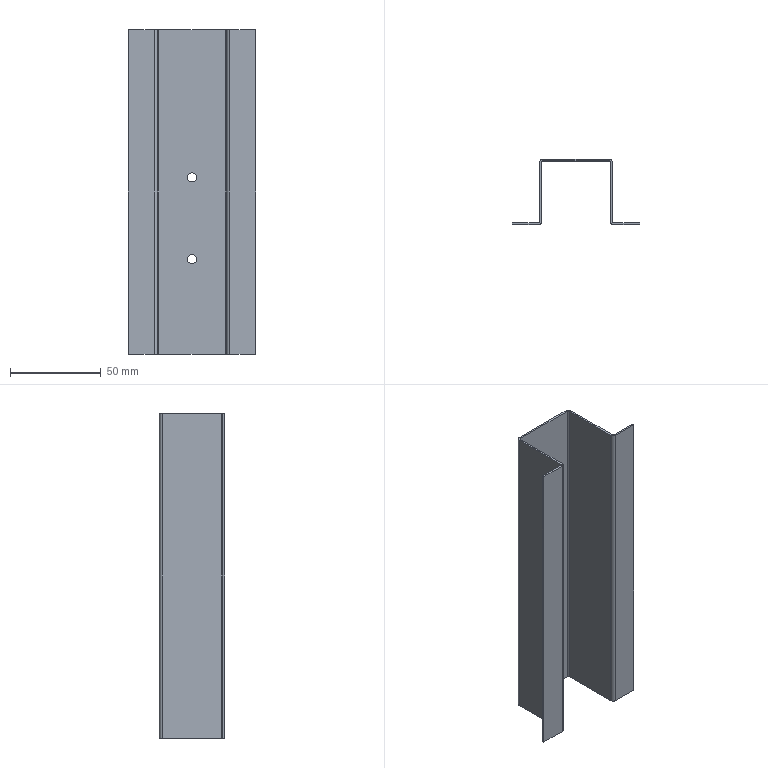Component | SolidWorks | CCQ-1.1-19Support1-1 | 1 solid | 34 faces | box 70 x 36 x 179 mm | volume 24641 mm3 | plane 22 | cylinder 12 | commonest cylinder face diameters 5 x4 1.473 x4 3.473 x4 | material 304
STEP:
#1=CARTESIAN_POINT('',(-2.067,-16.634,-3.327));
#2=VERTEX_POINT('',#1);
#3=CARTESIAN_POINT('',(-2.264,-16.634,-3.327));
#4=VERTEX_POINT('',#3);
#5=CARTESIAN_POINT('',(-2.165,-16.634,-3.327));
#6=DIRECTION('',(-0.,1.,0.));
#7=DIRECTION('',(-1.,0.,0.));
#8=AXIS2_PLACEMENT_3D('',#5,#6,#7);
#9=CIRCLE('',#8,0.09843);
#10=EDGE_CURVE('',#2,#4,#9,.T.);
#11=ORIENTED_EDGE('',*,*,#10,.F.);
#12=CARTESIAN_POINT('',(-2.067,-16.594,-3.327));
#13=VERTEX_POINT('',#12);
#14=CARTESIAN_POINT('',(-2.067,-16.988,-3.327));
#15=DIRECTION('',(-0.,1.,0.));
#16=VECTOR('',#15,39.37);
#17=LINE('',#14,#16);
#18=EDGE_CURVE('',#2,#13,#17,.T.);
#19=ORIENTED_EDGE('',*,*,#18,.T.);
#20=CARTESIAN_POINT('',(-2.264,-16.594,-3.327));
#21=VERTEX_POINT('',#20);
#22=CARTESIAN_POINT('',(-2.165,-16.594,-3.327));
#23=DIRECTION('',(-0.,1.,0.));
#24=DIRECTION('',(-1.,0.,0.));
#25=AXIS2_PLACEMENT_3D('',#22,#23,#24);
#26=CIRCLE('',#25,0.09843);
#27=EDGE_CURVE('',#13,#21,#26,.T.);
#28=ORIENTED_EDGE('',*,*,#27,.T.);
#29=CARTESIAN_POINT('',(-2.264,-16.988,-3.327));
#30=DIRECTION('',(-0.,1.,0.));
#31=VECTOR('',#30,39.37);
#32=LINE('',#29,#31);
#33=EDGE_CURVE('',#4,#21,#32,.T.);
#34=ORIENTED_EDGE('',*,*,#33,.F.);
#35=EDGE_LOOP('',(#11,#19,#28,#34));
#36=FACE_OUTER_BOUND('',#35,.T.);
#37=CARTESIAN_POINT('',(-2.165,-16.988,-3.327));
#38=DIRECTION('',(-0.,1.,0.));
#39=DIRECTION('',(-1.,0.,0.));
#40=AXIS2_PLACEMENT_3D('',#37,#38,#39);
#41=CYLINDRICAL_SURFACE('',#40,0.09843);
#42=ADVANCED_FACE('',(#36),#41,.F.);
#43=CARTESIAN_POINT('',(-2.067,-16.634,-5.098));
#44=VERTEX_POINT('',#43);
#45=CARTESIAN_POINT('',(-2.264,-16.634,-5.098));
#46=VERTEX_POINT('',#45);
#47=CARTESIAN_POINT('',(-2.165,-16.634,-5.098));
#48=DIRECTION('',(-0.,1.,0.));
#49=DIRECTION('',(-1.,0.,0.));
#50=AXIS2_PLACEMENT_3D('',#47,#48,#49);
#51=CIRCLE('',#50,0.09843);
#52=EDGE_CURVE('',#44,#46,#51,.T.);
#53=ORIENTED_EDGE('',*,*,#52,.F.);
#54=CARTESIAN_POINT('',(-2.067,-16.594,-5.098));
#55=VERTEX_POINT('',#54);
#56=CARTESIAN_POINT('',(-2.067,-16.988,-5.098));
#57=DIRECTION('',(-0.,1.,0.));
#58=VECTOR('',#57,39.37);
#59=LINE('',#56,#58);
#60=EDGE_CURVE('',#44,#55,#59,.T.);
#61=ORIENTED_EDGE('',*,*,#60,.T.);
#62=CARTESIAN_POINT('',(-2.264,-16.594,-5.098));
#63=VERTEX_POINT('',#62);
#64=CARTESIAN_POINT('',(-2.165,-16.594,-5.098));
#65=DIRECTION('',(-0.,1.,0.));
#66=DIRECTION('',(-1.,0.,0.));
#67=AXIS2_PLACEMENT_3D('',#64,#65,#66);
#68=CIRCLE('',#67,0.09843);
#69=EDGE_CURVE('',#55,#63,#68,.T.);
#70=ORIENTED_EDGE('',*,*,#69,.T.);
#71=CARTESIAN_POINT('',(-2.264,-16.988,-5.098));
#72=DIRECTION('',(-0.,1.,0.));
#73=VECTOR('',#72,39.37);
#74=LINE('',#71,#73);
#75=EDGE_CURVE('',#46,#63,#74,.T.);
#76=ORIENTED_EDGE('',*,*,#75,.F.);
#77=EDGE_LOOP('',(#53,#61,#70,#76));
#78=FACE_OUTER_BOUND('',#77,.T.);
#79=CARTESIAN_POINT('',(-2.165,-16.988,-5.098));
#80=DIRECTION('',(-0.,1.,0.));
#81=DIRECTION('',(-1.,0.,0.));
#82=AXIS2_PLACEMENT_3D('',#79,#80,#81);
#83=CYLINDRICAL_SURFACE('',#82,0.09843);
#84=ADVANCED_FACE('',(#78),#83,.F.);
#85=CARTESIAN_POINT('',(-2.982,-17.972,-7.165));
#86=VERTEX_POINT('',#85);
#87=CARTESIAN_POINT('',(-2.982,-18.012,-7.165));
#88=VERTEX_POINT('',#87);
#89=CARTESIAN_POINT('',(-2.982,-17.972,-7.165));
#90=DIRECTION('',(0.,-1.,0.));
#91=VECTOR('',#90,39.37);
#92=LINE('',#89,#91);
#93=EDGE_CURVE('',#86,#88,#92,.T.);
#94=ORIENTED_EDGE('',*,*,#93,.F.);
#95=CARTESIAN_POINT('',(-2.953,-17.943,-7.165));
#96=VERTEX_POINT('',#95);
#97=CARTESIAN_POINT('',(-2.982,-17.943,-7.165));
#98=DIRECTION('',(0.,0.,1.));
#99=DIRECTION('',(-1.,0.,0.));
#100=AXIS2_PLACEMENT_3D('',#97,#98,#99);
#101=CIRCLE('',#100,0.029);
#102=EDGE_CURVE('',#86,#96,#101,.T.);
#103=ORIENTED_EDGE('',*,*,#102,.T.);
#104=CARTESIAN_POINT('',(-2.913,-17.943,-7.165));
#105=VERTEX_POINT('',#104);
#106=CARTESIAN_POINT('',(-2.913,-17.943,-7.165));
#107=DIRECTION('',(-1.,0.,0.));
#108=VECTOR('',#107,39.37);
#109=LINE('',#106,#108);
#110=EDGE_CURVE('',#105,#96,#109,.T.);
#111=ORIENTED_EDGE('',*,*,#110,.F.);
#112=CARTESIAN_POINT('',(-2.982,-17.943,-7.165));
#113=DIRECTION('',(0.,0.,1.));
#114=DIRECTION('',(1.,0.,0.));
#115=AXIS2_PLACEMENT_3D('',#112,#113,#114);
#116=CIRCLE('',#115,0.06837);
#117=EDGE_CURVE('',#88,#105,#116,.T.);
#118=ORIENTED_EDGE('',*,*,#117,.F.);
#119=EDGE_LOOP('',(#94,#103,#111,#118));
#120=FACE_OUTER_BOUND('',#119,.T.);
#121=CARTESIAN_POINT('',(-2.982,-17.972,-7.165));
#122=DIRECTION('',(0.,0.,-1.));
#123=DIRECTION('',(-1.,0.,0.));
#124=AXIS2_PLACEMENT_3D('',#121,#122,#123);
#125=PLANE('',#124);
#126=ADVANCED_FACE('',(#120),#125,.T.);
#127=CARTESIAN_POINT('',(-3.543,-17.972,-7.165));
#128=VERTEX_POINT('',#127);
#129=CARTESIAN_POINT('',(-3.543,-17.972,-7.165));
#130=DIRECTION('',(1.,0.,0.));
#131=VECTOR('',#130,39.37);
#132=LINE('',#129,#131);
#133=EDGE_CURVE('',#128,#86,#132,.T.);
#134=ORIENTED_EDGE('',*,*,#133,.T.);
#135=ORIENTED_EDGE('',*,*,#93,.T.);
#136=CARTESIAN_POINT('',(-3.543,-18.012,-7.165));
#137=VERTEX_POINT('',#136);
#138=CARTESIAN_POINT('',(-3.543,-18.012,-7.165));
#139=DIRECTION('',(1.,0.,0.));
#140=VECTOR('',#139,39.37);
#141=LINE('',#138,#140);
#142=EDGE_CURVE('',#137,#88,#141,.T.);
#143=ORIENTED_EDGE('',*,*,#142,.F.);
#144=CARTESIAN_POINT('',(-3.543,-18.012,-7.165));
#145=DIRECTION('',(0.,1.,0.));
#146=VECTOR('',#145,39.37);
#147=LINE('',#144,#146);
#148=EDGE_CURVE('',#137,#128,#147,.T.);
#149=ORIENTED_EDGE('',*,*,#148,.T.);
#150=EDGE_LOOP('',(#134,#135,#143,#149));
#151=FACE_OUTER_BOUND('',#150,.T.);
#152=CARTESIAN_POINT('',(-2.913,-17.943,-7.165));
#153=DIRECTION('',(0.,0.,-1.));
#154=DIRECTION('',(-1.,0.,0.));
#155=AXIS2_PLACEMENT_3D('',#152,#153,#154);
#156=PLANE('',#155);
#157=ADVANCED_FACE('',(#151),#156,.T.);
#158=CARTESIAN_POINT('',(-2.953,-16.663,-7.165));
#159=VERTEX_POINT('',#158);
#160=CARTESIAN_POINT('',(-2.913,-16.663,-7.165));
#161=VERTEX_POINT('',#160);
#162=CARTESIAN_POINT('',(-2.953,-16.663,-7.165));
#163=DIRECTION('',(1.,0.,0.));
#164=VECTOR('',#163,39.37);
#165=LINE('',#162,#164);
#166=EDGE_CURVE('',#159,#161,#165,.T.);
#167=ORIENTED_EDGE('',*,*,#166,.F.);
#168=CARTESIAN_POINT('',(-2.884,-16.594,-7.165));
#169=VERTEX_POINT('',#168);
#170=CARTESIAN_POINT('',(-2.884,-16.663,-7.165));
#171=DIRECTION('',(0.,0.,-1.));
#172=DIRECTION('',(1.,0.,0.));
#173=AXIS2_PLACEMENT_3D('',#170,#171,#172);
#174=CIRCLE('',#173,0.06837);
#175=EDGE_CURVE('',#159,#169,#174,.T.);
#176=ORIENTED_EDGE('',*,*,#175,.T.);
#177=CARTESIAN_POINT('',(-2.884,-16.634,-7.165));
#178=VERTEX_POINT('',#177);
#179=CARTESIAN_POINT('',(-2.884,-16.634,-7.165));
#180=DIRECTION('',(0.,1.,0.));
#181=VECTOR('',#180,39.37);
#182=LINE('',#179,#181);
#183=EDGE_CURVE('',#178,#169,#182,.T.);
#184=ORIENTED_EDGE('',*,*,#183,.F.);
#185=CARTESIAN_POINT('',(-2.884,-16.663,-7.165));
#186=DIRECTION('',(0.,0.,-1.));
#187=DIRECTION('',(1.,0.,0.));
#188=AXIS2_PLACEMENT_3D('',#185,#186,#187);
#189=CIRCLE('',#188,0.029);
#190=EDGE_CURVE('',#161,#178,#189,.T.);
#191=ORIENTED_EDGE('',*,*,#190,.F.);
#192=EDGE_LOOP('',(#167,#176,#184,#191));
#193=FACE_OUTER_BOUND('',#192,.T.);
#194=CARTESIAN_POINT('',(-2.953,-16.663,-7.165));
#195=DIRECTION('',(0.,0.,-1.));
#196=DIRECTION('',(-1.,0.,0.));
#197=AXIS2_PLACEMENT_3D('',#194,#195,#196);
#198=PLANE('',#197);
#199=ADVANCED_FACE('',(#193),#198,.T.);
#200=CARTESIAN_POINT('',(-2.953,-17.972,-7.165));
#201=DIRECTION('',(0.,1.,0.));
#202=VECTOR('',#201,39.37);
#203=LINE('',#200,#202);
#204=EDGE_CURVE('',#96,#159,#203,.T.);
#205=ORIENTED_EDGE('',*,*,#204,.T.);
#206=ORIENTED_EDGE('',*,*,#166,.T.);
#207=CARTESIAN_POINT('',(-2.913,-17.972,-7.165));
#208=DIRECTION('',(0.,1.,0.));
#209=VECTOR('',#208,39.37);
#210=LINE('',#207,#209);
#211=EDGE_CURVE('',#105,#161,#210,.T.);
#212=ORIENTED_EDGE('',*,*,#211,.F.);
#213=ORIENTED_EDGE('',*,*,#110,.T.);
#214=EDGE_LOOP('',(#205,#206,#212,#213));
#215=FACE_OUTER_BOUND('',#214,.T.);
#216=CARTESIAN_POINT('',(-2.884,-16.634,-7.165));
#217=DIRECTION('',(0.,0.,-1.));
#218=DIRECTION('',(-1.,0.,0.));
#219=AXIS2_PLACEMENT_3D('',#216,#217,#218);
#220=PLANE('',#219);
#221=ADVANCED_FACE('',(#215),#220,.T.);
#222=CARTESIAN_POINT('',(-1.446,-16.594,-7.165));
#223=VERTEX_POINT('',#222);
#224=CARTESIAN_POINT('',(-1.446,-16.634,-7.165));
#225=VERTEX_POINT('',#224);
#226=CARTESIAN_POINT('',(-1.446,-16.594,-7.165));
#227=DIRECTION('',(0.,-1.,0.));
#228=VECTOR('',#227,39.37);
#229=LINE('',#226,#228);
#230=EDGE_CURVE('',#223,#225,#229,.T.);
#231=ORIENTED_EDGE('',*,*,#230,.F.);
#232=CARTESIAN_POINT('',(-1.378,-16.663,-7.165));
#233=VERTEX_POINT('',#232);
#234=CARTESIAN_POINT('',(-1.446,-16.663,-7.165));
#235=DIRECTION('',(0.,0.,-1.));
#236=DIRECTION('',(1.,0.,0.));
#237=AXIS2_PLACEMENT_3D('',#234,#235,#236);
#238=CIRCLE('',#237,0.06837);
#239=EDGE_CURVE('',#223,#233,#238,.T.);
#240=ORIENTED_EDGE('',*,*,#239,.T.);
#241=CARTESIAN_POINT('',(-1.417,-16.663,-7.165));
#242=VERTEX_POINT('',#241);
#243=CARTESIAN_POINT('',(-1.417,-16.663,-7.165));
#244=DIRECTION('',(1.,0.,0.));
#245=VECTOR('',#244,39.37);
#246=LINE('',#243,#245);
#247=EDGE_CURVE('',#242,#233,#246,.T.);
#248=ORIENTED_EDGE('',*,*,#247,.F.);
#249=CARTESIAN_POINT('',(-1.446,-16.663,-7.165));
#250=DIRECTION('',(0.,0.,-1.));
#251=DIRECTION('',(1.,0.,0.));
#252=AXIS2_PLACEMENT_3D('',#249,#250,#251);
#253=CIRCLE('',#252,0.029);
#254=EDGE_CURVE('',#225,#242,#253,.T.);
#255=ORIENTED_EDGE('',*,*,#254,.F.);
#256=EDGE_LOOP('',(#231,#240,#248,#255));
#257=FACE_OUTER_BOUND('',#256,.T.);
#258=CARTESIAN_POINT('',(-1.446,-16.594,-7.165));
#259=DIRECTION('',(0.,0.,-1.));
#260=DIRECTION('',(-1.,0.,0.));
#261=AXIS2_PLACEMENT_3D('',#258,#259,#260);
#262=PLANE('',#261);
#263=ADVANCED_FACE('',(#257),#262,.T.);
#264=CARTESIAN_POINT('',(-2.953,-16.594,-7.165));
#265=DIRECTION('',(1.,0.,0.));
#266=VECTOR('',#265,39.37);
#267=LINE('',#264,#266);
#268=EDGE_CURVE('',#169,#223,#267,.T.);
#269=ORIENTED_EDGE('',*,*,#268,.T.);
#270=ORIENTED_EDGE('',*,*,#230,.T.);
#271=CARTESIAN_POINT('',(-2.953,-16.634,-7.165));
#272=DIRECTION('',(1.,0.,0.));
#273=VECTOR('',#272,39.37);
#274=LINE('',#271,#273);
#275=EDGE_CURVE('',#178,#225,#274,.T.);
#276=ORIENTED_EDGE('',*,*,#275,.F.);
#277=ORIENTED_EDGE('',*,*,#183,.T.);
#278=EDGE_LOOP('',(#269,#270,#276,#277));
#279=FACE_OUTER_BOUND('',#278,.T.);
#280=CARTESIAN_POINT('',(-1.417,-16.663,-7.165));
#281=DIRECTION('',(0.,0.,-1.));
#282=DIRECTION('',(-1.,0.,0.));
#283=AXIS2_PLACEMENT_3D('',#280,#281,#282);
#284=PLANE('',#283);
#285=ADVANCED_FACE('',(#279),#284,.T.);
#286=CARTESIAN_POINT('',(-1.378,-17.943,-7.165));
#287=VERTEX_POINT('',#286);
#288=CARTESIAN_POINT('',(-1.417,-17.943,-7.165));
#289=VERTEX_POINT('',#288);
#290=CARTESIAN_POINT('',(-1.378,-17.943,-7.165));
#291=DIRECTION('',(-1.,-0.,0.));
#292=VECTOR('',#291,39.37);
#293=LINE('',#290,#292);
#294=EDGE_CURVE('',#287,#289,#293,.T.);
#295=ORIENTED_EDGE('',*,*,#294,.F.);
#296=CARTESIAN_POINT('',(-1.349,-17.972,-7.165));
#297=VERTEX_POINT('',#296);
#298=CARTESIAN_POINT('',(-1.349,-17.943,-7.165));
#299=DIRECTION('',(0.,0.,1.));
#300=DIRECTION('',(-1.,-0.,0.));
#301=AXIS2_PLACEMENT_3D('',#298,#299,#300);
#302=CIRCLE('',#301,0.029);
#303=EDGE_CURVE('',#287,#297,#302,.T.);
#304=ORIENTED_EDGE('',*,*,#303,.T.);
#305=CARTESIAN_POINT('',(-1.349,-18.012,-7.165));
#306=VERTEX_POINT('',#305);
#307=CARTESIAN_POINT('',(-1.349,-18.012,-7.165));
#308=DIRECTION('',(0.,1.,0.));
#309=VECTOR('',#308,39.37);
#310=LINE('',#307,#309);
#311=EDGE_CURVE('',#306,#297,#310,.T.);
#312=ORIENTED_EDGE('',*,*,#311,.F.);
#313=CARTESIAN_POINT('',(-1.349,-17.943,-7.165));
#314=DIRECTION('',(0.,0.,1.));
#315=DIRECTION('',(1.,0.,0.));
#316=AXIS2_PLACEMENT_3D('',#313,#314,#315);
#317=CIRCLE('',#316,0.06837);
#318=EDGE_CURVE('',#289,#306,#317,.T.);
#319=ORIENTED_EDGE('',*,*,#318,.F.);
#320=EDGE_LOOP('',(#295,#304,#312,#319));
#321=FACE_OUTER_BOUND('',#320,.T.);
#322=CARTESIAN_POINT('',(-1.378,-17.943,-7.165));
#323=DIRECTION('',(0.,0.,-1.));
#324=DIRECTION('',(-1.,0.,0.));
#325=AXIS2_PLACEMENT_3D('',#322,#323,#324);
#326=PLANE('',#325);
#327=ADVANCED_FACE('',(#321),#326,.T.);
#328=CARTESIAN_POINT('',(-1.378,-16.594,-7.165));
#329=DIRECTION('',(0.,-1.,0.));
#330=VECTOR('',#329,39.37);
#331=LINE('',#328,#330);
#332=EDGE_CURVE('',#233,#287,#331,.T.);
#333=ORIENTED_EDGE('',*,*,#332,.T.);
#334=ORIENTED_EDGE('',*,*,#294,.T.);
#335=CARTESIAN_POINT('',(-1.417,-16.594,-7.165));
#336=DIRECTION('',(0.,-1.,0.));
#337=VECTOR('',#336,39.37);
#338=LINE('',#335,#337);
#339=EDGE_CURVE('',#242,#289,#338,.T.);
#340=ORIENTED_EDGE('',*,*,#339,.F.);
#341=ORIENTED_EDGE('',*,*,#247,.T.);
#342=EDGE_LOOP('',(#333,#334,#340,#341));
#343=FACE_OUTER_BOUND('',#342,.T.);
#344=CARTESIAN_POINT('',(-1.349,-18.012,-7.165));
#345=DIRECTION('',(0.,0.,-1.));
#346=DIRECTION('',(-1.,0.,0.));
#347=AXIS2_PLACEMENT_3D('',#344,#345,#346);
#348=PLANE('',#347);
#349=ADVANCED_FACE('',(#343),#348,.T.);
#350=CARTESIAN_POINT('',(-0.7874,-18.012,-0.1181));
#351=VERTEX_POINT('',#350);
#352=CARTESIAN_POINT('',(-0.7874,-18.012,-7.165));
#353=VERTEX_POINT('',#352);
#354=CARTESIAN_POINT('',(-0.7874,-18.012,-0.07874));
#355=DIRECTION('',(0.,0.,-1.));
#356=VECTOR('',#355,39.37);
#357=LINE('',#354,#356);
#358=EDGE_CURVE('',#351,#353,#357,.T.);
#359=ORIENTED_EDGE('',*,*,#358,.F.);
#360=CARTESIAN_POINT('',(-1.349,-18.012,-0.1181));
#361=VERTEX_POINT('',#360);
#362=CARTESIAN_POINT('',(-1.378,-18.012,-0.1181));
#363=DIRECTION('',(-1.,0.,0.));
#364=VECTOR('',#363,39.37);
#365=LINE('',#362,#364);
#366=EDGE_CURVE('',#351,#361,#365,.T.);
#367=ORIENTED_EDGE('',*,*,#366,.T.);
#368=CARTESIAN_POINT('',(-1.349,-18.012,-0.07874));
#369=DIRECTION('',(0.,0.,-1.));
#370=VECTOR('',#369,39.37);
#371=LINE('',#368,#370);
#372=EDGE_CURVE('',#361,#306,#371,.T.);
#373=ORIENTED_EDGE('',*,*,#372,.T.);
#374=CARTESIAN_POINT('',(-1.378,-18.012,-7.165));
#375=DIRECTION('',(1.,-0.,0.));
#376=VECTOR('',#375,39.37);
#377=LINE('',#374,#376);
#378=EDGE_CURVE('',#306,#353,#377,.T.);
#379=ORIENTED_EDGE('',*,*,#378,.T.);
#380=EDGE_LOOP('',(#359,#367,#373,#379));
#381=FACE_OUTER_BOUND('',#380,.T.);
#382=CARTESIAN_POINT('',(-1.378,-18.012,-0.07874));
#383=DIRECTION('',(0.,1.,0.));
#384=DIRECTION('',(-1.,0.,0.));
#385=AXIS2_PLACEMENT_3D('',#382,#383,#384);
#386=PLANE('',#385);
#387=ADVANCED_FACE('',(#381),#386,.F.);
#388=CARTESIAN_POINT('',(-0.7874,-17.972,-0.1181));
#389=VERTEX_POINT('',#388);
#390=CARTESIAN_POINT('',(-0.7874,-17.972,-0.1181));
#391=DIRECTION('',(0.,1.,0.));
#392=VECTOR('',#391,39.37);
#393=LINE('',#390,#392);
#394=EDGE_CURVE('',#351,#389,#393,.T.);
#395=ORIENTED_EDGE('',*,*,#394,.F.);
#396=ORIENTED_EDGE('',*,*,#358,.T.);
#397=CARTESIAN_POINT('',(-0.7874,-17.972,-7.165));
#398=VERTEX_POINT('',#397);
#399=CARTESIAN_POINT('',(-0.7874,-17.972,-7.165));
#400=DIRECTION('',(0.,-1.,0.));
#401=VECTOR('',#400,39.37);
#402=LINE('',#399,#401);
#403=EDGE_CURVE('',#398,#353,#402,.T.);
#404=ORIENTED_EDGE('',*,*,#403,.F.);
#405=CARTESIAN_POINT('',(-0.7874,-17.972,-0.07874));
#406=DIRECTION('',(0.,0.,-1.));
#407=VECTOR('',#406,39.37);
#408=LINE('',#405,#407);
#409=EDGE_CURVE('',#389,#398,#408,.T.);
#410=ORIENTED_EDGE('',*,*,#409,.F.);
#411=EDGE_LOOP('',(#395,#396,#404,#410));
#412=FACE_OUTER_BOUND('',#411,.T.);
#413=CARTESIAN_POINT('',(-0.7874,-17.972,-0.07874));
#414=DIRECTION('',(1.,0.,0.));
#415=DIRECTION('',(0.,0.,-1.));
#416=AXIS2_PLACEMENT_3D('',#413,#414,#415);
#417=PLANE('',#416);
#418=ADVANCED_FACE('',(#412),#417,.T.);
#419=CARTESIAN_POINT('',(-1.349,-17.972,-0.1181));
#420=VERTEX_POINT('',#419);
#421=CARTESIAN_POINT('',(-1.378,-17.972,-0.1181));
#422=DIRECTION('',(-1.,0.,0.));
#423=VECTOR('',#422,39.37);
#424=LINE('',#421,#423);
#425=EDGE_CURVE('',#389,#420,#424,.T.);
#426=ORIENTED_EDGE('',*,*,#425,.F.);
#427=ORIENTED_EDGE('',*,*,#409,.T.);
#428=CARTESIAN_POINT('',(-1.378,-17.972,-7.165));
#429=DIRECTION('',(1.,-0.,0.));
#430=VECTOR('',#429,39.37);
#431=LINE('',#428,#430);
#432=EDGE_CURVE('',#297,#398,#431,.T.);
#433=ORIENTED_EDGE('',*,*,#432,.F.);
#434=CARTESIAN_POINT('',(-1.349,-17.972,-0.07874));
#435=DIRECTION('',(0.,0.,-1.));
#436=VECTOR('',#435,39.37);
#437=LINE('',#434,#436);
#438=EDGE_CURVE('',#420,#297,#437,.T.);
#439=ORIENTED_EDGE('',*,*,#438,.F.);
#440=EDGE_LOOP('',(#426,#427,#433,#439));
#441=FACE_OUTER_BOUND('',#440,.T.);
#442=CARTESIAN_POINT('',(-1.378,-17.972,-0.07874));
#443=DIRECTION('',(0.,1.,0.));
#444=DIRECTION('',(-1.,0.,0.));
#445=AXIS2_PLACEMENT_3D('',#442,#443,#444);
#446=PLANE('',#445);
#447=ADVANCED_FACE('',(#441),#446,.T.);
#448=CARTESIAN_POINT('',(-1.378,-17.943,-0.1181));
#449=VERTEX_POINT('',#448);
#450=CARTESIAN_POINT('',(-1.349,-17.943,-0.1181));
#451=DIRECTION('',(0.,0.,-1.));
#452=DIRECTION('',(-1.,0.,0.));
#453=AXIS2_PLACEMENT_3D('',#450,#451,#452);
#454=CIRCLE('',#453,0.029);
#455=EDGE_CURVE('',#420,#449,#454,.T.);
#456=ORIENTED_EDGE('',*,*,#455,.F.);
#457=ORIENTED_EDGE('',*,*,#438,.T.);
#458=ORIENTED_EDGE('',*,*,#303,.F.);
#459=CARTESIAN_POINT('',(-1.378,-17.943,-0.07874));
#460=DIRECTION('',(0.,0.,-1.));
#461=VECTOR('',#460,39.37);
#462=LINE('',#459,#461);
#463=EDGE_CURVE('',#449,#287,#462,.T.);
#464=ORIENTED_EDGE('',*,*,#463,.F.);
#465=EDGE_LOOP('',(#456,#457,#458,#464));
#466=FACE_OUTER_BOUND('',#465,.T.);
#467=CARTESIAN_POINT('',(-1.349,-17.943,-0.07874));
#468=DIRECTION('',(0.,0.,-1.));
#469=DIRECTION('',(-1.,0.,0.));
#470=AXIS2_PLACEMENT_3D('',#467,#468,#469);
#471=CYLINDRICAL_SURFACE('',#470,0.029);
#472=ADVANCED_FACE('',(#466),#471,.F.);
#473=CARTESIAN_POINT('',(-1.378,-16.663,-0.1181));
#474=VERTEX_POINT('',#473);
#475=CARTESIAN_POINT('',(-1.378,-16.594,-0.1181));
#476=DIRECTION('',(-0.,1.,0.));
#477=VECTOR('',#476,39.37);
#478=LINE('',#475,#477);
#479=EDGE_CURVE('',#449,#474,#478,.T.);
#480=ORIENTED_EDGE('',*,*,#479,.F.);
#481=ORIENTED_EDGE('',*,*,#463,.T.);
#482=ORIENTED_EDGE('',*,*,#332,.F.);
#483=CARTESIAN_POINT('',(-1.378,-16.663,-0.07874));
#484=DIRECTION('',(0.,0.,-1.));
#485=VECTOR('',#484,39.37);
#486=LINE('',#483,#485);
#487=EDGE_CURVE('',#474,#233,#486,.T.);
#488=ORIENTED_EDGE('',*,*,#487,.F.);
#489=EDGE_LOOP('',(#480,#481,#482,#488));
#490=FACE_OUTER_BOUND('',#489,.T.);
#491=CARTESIAN_POINT('',(-1.378,-16.594,-0.07874));
#492=DIRECTION('',(1.,0.,0.));
#493=DIRECTION('',(-0.,1.,0.));
#494=AXIS2_PLACEMENT_3D('',#491,#492,#493);
#495=PLANE('',#494);
#496=ADVANCED_FACE('',(#490),#495,.T.);
#497=CARTESIAN_POINT('',(-1.446,-16.594,-0.1181));
#498=VERTEX_POINT('',#497);
#499=CARTESIAN_POINT('',(-1.446,-16.663,-0.1181));
#500=DIRECTION('',(0.,0.,1.));
#501=DIRECTION('',(-1.,0.,0.));
#502=AXIS2_PLACEMENT_3D('',#499,#500,#501);
#503=CIRCLE('',#502,0.06837);
#504=EDGE_CURVE('',#474,#498,#503,.T.);
#505=ORIENTED_EDGE('',*,*,#504,.F.);
#506=ORIENTED_EDGE('',*,*,#487,.T.);
#507=ORIENTED_EDGE('',*,*,#239,.F.);
#508=CARTESIAN_POINT('',(-1.446,-16.594,-0.07874));
#509=DIRECTION('',(0.,0.,-1.));
#510=VECTOR('',#509,39.37);
#511=LINE('',#508,#510);
#512=EDGE_CURVE('',#498,#223,#511,.T.);
#513=ORIENTED_EDGE('',*,*,#512,.F.);
#514=EDGE_LOOP('',(#505,#506,#507,#513));
#515=FACE_OUTER_BOUND('',#514,.T.);
#516=CARTESIAN_POINT('',(-1.446,-16.663,-0.07874));
#517=DIRECTION('',(0.,0.,-1.));
#518=DIRECTION('',(-1.,0.,0.));
#519=AXIS2_PLACEMENT_3D('',#516,#517,#518);
#520=CYLINDRICAL_SURFACE('',#519,0.06837);
#521=ADVANCED_FACE('',(#515),#520,.T.);
#522=CARTESIAN_POINT('',(-2.884,-16.594,-0.1181));
#523=VERTEX_POINT('',#522);
#524=CARTESIAN_POINT('',(-2.953,-16.594,-0.1181));
#525=DIRECTION('',(-1.,-0.,0.));
#526=VECTOR('',#525,39.37);
#527=LINE('',#524,#526);
#528=EDGE_CURVE('',#498,#523,#527,.T.);
#529=ORIENTED_EDGE('',*,*,#528,.F.);
#530=ORIENTED_EDGE('',*,*,#512,.T.);
#531=ORIENTED_EDGE('',*,*,#268,.F.);
#532=CARTESIAN_POINT('',(-2.884,-16.594,-0.07874));
#533=DIRECTION('',(0.,0.,-1.));
#534=VECTOR('',#533,39.37);
#535=LINE('',#532,#534);
#536=EDGE_CURVE('',#523,#169,#535,.T.);
#537=ORIENTED_EDGE('',*,*,#536,.F.);
#538=EDGE_LOOP('',(#529,#530,#531,#537));
#539=FACE_OUTER_BOUND('',#538,.T.);
#540=CARTESIAN_POINT('',(-2.165,-16.594,-3.327));
#541=DIRECTION('',(-0.,1.,0.));
#542=DIRECTION('',(-1.,0.,0.));
#543=AXIS2_PLACEMENT_3D('',#540,#541,#542);
#544=CIRCLE('',#543,0.09843);
#545=EDGE_CURVE('',#21,#13,#544,.T.);
#546=ORIENTED_EDGE('',*,*,#545,.F.);
#547=ORIENTED_EDGE('',*,*,#27,.F.);
#548=EDGE_LOOP('',(#546,#547));
#549=FACE_BOUND('',#548,.T.);
#550=CARTESIAN_POINT('',(-2.165,-16.594,-5.098));
#551=DIRECTION('',(-0.,1.,0.));
#552=DIRECTION('',(-1.,0.,0.));
#553=AXIS2_PLACEMENT_3D('',#550,#551,#552);
#554=CIRCLE('',#553,0.09843);
#555=EDGE_CURVE('',#63,#55,#554,.T.);
#556=ORIENTED_EDGE('',*,*,#555,.F.);
#557=ORIENTED_EDGE('',*,*,#69,.F.);
#558=EDGE_LOOP('',(#556,#557));
#559=FACE_BOUND('',#558,.T.);
#560=CARTESIAN_POINT('',(-2.953,-16.594,-0.07874));
#561=DIRECTION('',(-0.,1.,0.));
#562=DIRECTION('',(-1.,-0.,0.));
#563=AXIS2_PLACEMENT_3D('',#560,#561,#562);
#564=PLANE('',#563);
#565=ADVANCED_FACE('',(#539,#549,#559),#564,.T.);
#566=CARTESIAN_POINT('',(-2.953,-16.663,-0.1181));
#567=VERTEX_POINT('',#566);
#568=CARTESIAN_POINT('',(-2.884,-16.663,-0.1181));
#569=DIRECTION('',(0.,0.,1.));
#570=DIRECTION('',(-1.,0.,0.));
#571=AXIS2_PLACEMENT_3D('',#568,#569,#570);
#572=CIRCLE('',#571,0.06837);
#573=EDGE_CURVE('',#523,#567,#572,.T.);
#574=ORIENTED_EDGE('',*,*,#573,.F.);
#575=ORIENTED_EDGE('',*,*,#536,.T.);
#576=ORIENTED_EDGE('',*,*,#175,.F.);
#577=CARTESIAN_POINT('',(-2.953,-16.663,-0.07874));
#578=DIRECTION('',(0.,0.,-1.));
#579=VECTOR('',#578,39.37);
#580=LINE('',#577,#579);
#581=EDGE_CURVE('',#567,#159,#580,.T.);
#582=ORIENTED_EDGE('',*,*,#581,.F.);
#583=EDGE_LOOP('',(#574,#575,#576,#582));
#584=FACE_OUTER_BOUND('',#583,.T.);
#585=CARTESIAN_POINT('',(-2.884,-16.663,-0.07874));
#586=DIRECTION('',(0.,0.,-1.));
#587=DIRECTION('',(-1.,0.,0.));
#588=AXIS2_PLACEMENT_3D('',#585,#586,#587);
#589=CYLINDRICAL_SURFACE('',#588,0.06837);
#590=ADVANCED_FACE('',(#584),#589,.T.);
#591=CARTESIAN_POINT('',(-2.953,-17.943,-0.1181));
#592=VERTEX_POINT('',#591);
#593=CARTESIAN_POINT('',(-2.953,-17.972,-0.1181));
#594=DIRECTION('',(0.,-1.,0.));
#595=VECTOR('',#594,39.37);
#596=LINE('',#593,#595);
#597=EDGE_CURVE('',#567,#592,#596,.T.);
#598=ORIENTED_EDGE('',*,*,#597,.F.);
#599=ORIENTED_EDGE('',*,*,#581,.T.);
#600=ORIENTED_EDGE('',*,*,#204,.F.);
#601=CARTESIAN_POINT('',(-2.953,-17.943,-0.07874));
#602=DIRECTION('',(0.,0.,-1.));
#603=VECTOR('',#602,39.37);
#604=LINE('',#601,#603);
#605=EDGE_CURVE('',#592,#96,#604,.T.);
#606=ORIENTED_EDGE('',*,*,#605,.F.);
#607=EDGE_LOOP('',(#598,#599,#600,#606));
#608=FACE_OUTER_BOUND('',#607,.T.);
#609=CARTESIAN_POINT('',(-2.953,-17.972,-0.07874));
#610=DIRECTION('',(-1.,0.,0.));
#611=DIRECTION('',(0.,0.,1.));
#612=AXIS2_PLACEMENT_3D('',#609,#610,#611);
#613=PLANE('',#612);
#614=ADVANCED_FACE('',(#608),#613,.T.);
#615=CARTESIAN_POINT('',(-2.982,-17.972,-0.1181));
#616=VERTEX_POINT('',#615);
#617=CARTESIAN_POINT('',(-2.982,-17.943,-0.1181));
#618=DIRECTION('',(0.,0.,-1.));
#619=DIRECTION('',(-1.,0.,0.));
#620=AXIS2_PLACEMENT_3D('',#617,#618,#619);
#621=CIRCLE('',#620,0.029);
#622=EDGE_CURVE('',#592,#616,#621,.T.);
#623=ORIENTED_EDGE('',*,*,#622,.F.);
#624=ORIENTED_EDGE('',*,*,#605,.T.);
#625=ORIENTED_EDGE('',*,*,#102,.F.);
#626=CARTESIAN_POINT('',(-2.982,-17.972,-0.07874));
#627=DIRECTION('',(0.,0.,-1.));
#628=VECTOR('',#627,39.37);
#629=LINE('',#626,#628);
#630=EDGE_CURVE('',#616,#86,#629,.T.);
#631=ORIENTED_EDGE('',*,*,#630,.F.);
#632=EDGE_LOOP('',(#623,#624,#625,#631));
#633=FACE_OUTER_BOUND('',#632,.T.);
#634=CARTESIAN_POINT('',(-2.982,-17.943,-0.07874));
#635=DIRECTION('',(0.,0.,-1.));
#636=DIRECTION('',(-1.,0.,0.));
#637=AXIS2_PLACEMENT_3D('',#634,#635,#636);
#638=CYLINDRICAL_SURFACE('',#637,0.029);
#639=ADVANCED_FACE('',(#633),#638,.F.);
#640=CARTESIAN_POINT('',(-3.543,-17.972,-0.1181));
#641=VERTEX_POINT('',#640);
#642=CARTESIAN_POINT('',(-3.543,-17.972,-0.1181));
#643=DIRECTION('',(-1.,0.,0.));
#644=VECTOR('',#643,39.37);
#645=LINE('',#642,#644);
#646=EDGE_CURVE('',#616,#641,#645,.T.);
#647=ORIENTED_EDGE('',*,*,#646,.F.);
#648=ORIENTED_EDGE('',*,*,#630,.T.);
#649=ORIENTED_EDGE('',*,*,#133,.F.);
#650=CARTESIAN_POINT('',(-3.543,-17.972,-0.07874));
#651=DIRECTION('',(0.,0.,-1.));
#652=VECTOR('',#651,39.37);
#653=LINE('',#650,#652);
#654=EDGE_CURVE('',#641,#128,#653,.T.);
#655=ORIENTED_EDGE('',*,*,#654,.F.);
#656=EDGE_LOOP('',(#647,#648,#649,#655));
#657=FACE_OUTER_BOUND('',#656,.T.);
#658=CARTESIAN_POINT('',(-3.543,-17.972,-0.07874));
#659=DIRECTION('',(0.,1.,0.));
#660=DIRECTION('',(0.,0.,1.));
#661=AXIS2_PLACEMENT_3D('',#658,#659,#660);
#662=PLANE('',#661);
#663=ADVANCED_FACE('',(#657),#662,.T.);
#664=CARTESIAN_POINT('',(-3.543,-18.012,-0.1181));
#665=VERTEX_POINT('',#664);
#666=CARTESIAN_POINT('',(-3.543,-18.012,-0.1181));
#667=DIRECTION('',(0.,-1.,0.));
#668=VECTOR('',#667,39.37);
#669=LINE('',#666,#668);
#670=EDGE_CURVE('',#641,#665,#669,.T.);
#671=ORIENTED_EDGE('',*,*,#670,.F.);
#672=ORIENTED_EDGE('',*,*,#654,.T.);
#673=ORIENTED_EDGE('',*,*,#148,.F.);
#674=CARTESIAN_POINT('',(-3.543,-18.012,-0.07874));
#675=DIRECTION('',(0.,0.,-1.));
#676=VECTOR('',#675,39.37);
#677=LINE('',#674,#676);
#678=EDGE_CURVE('',#665,#137,#677,.T.);
#679=ORIENTED_EDGE('',*,*,#678,.F.);
#680=EDGE_LOOP('',(#671,#672,#673,#679));
#681=FACE_OUTER_BOUND('',#680,.T.);
#682=CARTESIAN_POINT('',(-3.543,-18.012,-0.07874));
#683=DIRECTION('',(-1.,0.,0.));
#684=DIRECTION('',(0.,0.,1.));
#685=AXIS2_PLACEMENT_3D('',#682,#683,#684);
#686=PLANE('',#685);
#687=ADVANCED_FACE('',(#681),#686,.T.);
#688=CARTESIAN_POINT('',(-2.982,-18.012,-0.1181));
#689=VERTEX_POINT('',#688);
#690=CARTESIAN_POINT('',(-2.982,-18.012,-0.07874));
#691=DIRECTION('',(0.,0.,-1.));
#692=VECTOR('',#691,39.37);
#693=LINE('',#690,#692);
#694=EDGE_CURVE('',#689,#88,#693,.T.);
#695=ORIENTED_EDGE('',*,*,#694,.F.);
#696=CARTESIAN_POINT('',(-3.543,-18.012,-0.1181));
#697=DIRECTION('',(-1.,0.,0.));
#698=VECTOR('',#697,39.37);
#699=LINE('',#696,#698);
#700=EDGE_CURVE('',#689,#665,#699,.T.);
#701=ORIENTED_EDGE('',*,*,#700,.T.);
#702=ORIENTED_EDGE('',*,*,#678,.T.);
#703=ORIENTED_EDGE('',*,*,#142,.T.);
#704=EDGE_LOOP('',(#695,#701,#702,#703));
#705=FACE_OUTER_BOUND('',#704,.T.);
#706=CARTESIAN_POINT('',(-3.543,-18.012,-0.07874));
#707=DIRECTION('',(0.,1.,0.));
#708=DIRECTION('',(0.,0.,1.));
#709=AXIS2_PLACEMENT_3D('',#706,#707,#708);
#710=PLANE('',#709);
#711=ADVANCED_FACE('',(#705),#710,.F.);
#712=CARTESIAN_POINT('',(-2.913,-17.943,-0.1181));
#713=VERTEX_POINT('',#712);
#714=CARTESIAN_POINT('',(-2.913,-17.943,-0.07874));
#715=DIRECTION('',(0.,0.,-1.));
#716=VECTOR('',#715,39.37);
#717=LINE('',#714,#716);
#718=EDGE_CURVE('',#713,#105,#717,.T.);
#719=ORIENTED_EDGE('',*,*,#718,.F.);
#720=CARTESIAN_POINT('',(-2.982,-17.943,-0.1181));
#721=DIRECTION('',(0.,0.,-1.));
#722=DIRECTION('',(-1.,0.,0.));
#723=AXIS2_PLACEMENT_3D('',#720,#721,#722);
#724=CIRCLE('',#723,0.06837);
#725=EDGE_CURVE('',#713,#689,#724,.T.);
#726=ORIENTED_EDGE('',*,*,#725,.T.);
#727=ORIENTED_EDGE('',*,*,#694,.T.);
#728=ORIENTED_EDGE('',*,*,#117,.T.);
#729=EDGE_LOOP('',(#719,#726,#727,#728));
#730=FACE_OUTER_BOUND('',#729,.T.);
#731=CARTESIAN_POINT('',(-2.982,-17.943,-0.07874));
#732=DIRECTION('',(0.,0.,-1.));
#733=DIRECTION('',(-1.,0.,0.));
#734=AXIS2_PLACEMENT_3D('',#731,#732,#733);
#735=CYLINDRICAL_SURFACE('',#734,0.06837);
#736=ADVANCED_FACE('',(#730),#735,.T.);
#737=CARTESIAN_POINT('',(-2.913,-16.663,-0.1181));
#738=VERTEX_POINT('',#737);
#739=CARTESIAN_POINT('',(-2.913,-16.663,-0.07874));
#740=DIRECTION('',(0.,0.,-1.));
#741=VECTOR('',#740,39.37);
#742=LINE('',#739,#741);
#743=EDGE_CURVE('',#738,#161,#742,.T.);
#744=ORIENTED_EDGE('',*,*,#743,.F.);
#745=CARTESIAN_POINT('',(-2.913,-17.972,-0.1181));
#746=DIRECTION('',(0.,-1.,0.));
#747=VECTOR('',#746,39.37);
#748=LINE('',#745,#747);
#749=EDGE_CURVE('',#738,#713,#748,.T.);
#750=ORIENTED_EDGE('',*,*,#749,.T.);
#751=ORIENTED_EDGE('',*,*,#718,.T.);
#752=ORIENTED_EDGE('',*,*,#211,.T.);
#753=EDGE_LOOP('',(#744,#750,#751,#752));
#754=FACE_OUTER_BOUND('',#753,.T.);
#755=CARTESIAN_POINT('',(-2.913,-17.972,-0.07874));
#756=DIRECTION('',(-1.,0.,0.));
#757=DIRECTION('',(0.,0.,1.));
#758=AXIS2_PLACEMENT_3D('',#755,#756,#757);
#759=PLANE('',#758);
#760=ADVANCED_FACE('',(#754),#759,.F.);
#761=CARTESIAN_POINT('',(-2.884,-16.634,-0.1181));
#762=VERTEX_POINT('',#761);
#763=CARTESIAN_POINT('',(-2.884,-16.634,-0.07874));
#764=DIRECTION('',(0.,0.,-1.));
#765=VECTOR('',#764,39.37);
#766=LINE('',#763,#765);
#767=EDGE_CURVE('',#762,#178,#766,.T.);
#768=ORIENTED_EDGE('',*,*,#767,.F.);
#769=CARTESIAN_POINT('',(-2.884,-16.663,-0.1181));
#770=DIRECTION('',(0.,0.,1.));
#771=DIRECTION('',(-1.,0.,0.));
#772=AXIS2_PLACEMENT_3D('',#769,#770,#771);
#773=CIRCLE('',#772,0.029);
#774=EDGE_CURVE('',#762,#738,#773,.T.);
#775=ORIENTED_EDGE('',*,*,#774,.T.);
#776=ORIENTED_EDGE('',*,*,#743,.T.);
#777=ORIENTED_EDGE('',*,*,#190,.T.);
#778=EDGE_LOOP('',(#768,#775,#776,#777));
#779=FACE_OUTER_BOUND('',#778,.T.);
#780=CARTESIAN_POINT('',(-2.884,-16.663,-0.07874));
#781=DIRECTION('',(0.,0.,-1.));
#782=DIRECTION('',(-1.,0.,0.));
#783=AXIS2_PLACEMENT_3D('',#780,#781,#782);
#784=CYLINDRICAL_SURFACE('',#783,0.029);
#785=ADVANCED_FACE('',(#779),#784,.F.);
#786=CARTESIAN_POINT('',(-2.165,-16.634,-3.327));
#787=DIRECTION('',(-0.,1.,0.));
#788=DIRECTION('',(-1.,0.,0.));
#789=AXIS2_PLACEMENT_3D('',#786,#787,#788);
#790=CIRCLE('',#789,0.09843);
#791=EDGE_CURVE('',#4,#2,#790,.T.);
#792=ORIENTED_EDGE('',*,*,#791,.T.);
#793=ORIENTED_EDGE('',*,*,#10,.T.);
#794=EDGE_LOOP('',(#792,#793));
#795=FACE_BOUND('',#794,.T.);
#796=CARTESIAN_POINT('',(-2.165,-16.634,-5.098));
#797=DIRECTION('',(-0.,1.,0.));
#798=DIRECTION('',(-1.,0.,0.));
#799=AXIS2_PLACEMENT_3D('',#796,#797,#798);
#800=CIRCLE('',#799,0.09843);
#801=EDGE_CURVE('',#46,#44,#800,.T.);
#802=ORIENTED_EDGE('',*,*,#801,.T.);
#803=ORIENTED_EDGE('',*,*,#52,.T.);
#804=EDGE_LOOP('',(#802,#803));
#805=FACE_BOUND('',#804,.T.);
#806=CARTESIAN_POINT('',(-1.446,-16.634,-0.1181));
#807=VERTEX_POINT('',#806);
#808=CARTESIAN_POINT('',(-1.446,-16.634,-0.07874));
#809=DIRECTION('',(0.,0.,-1.));
#810=VECTOR('',#809,39.37);
#811=LINE('',#808,#810);
#812=EDGE_CURVE('',#807,#225,#811,.T.);
#813=ORIENTED_EDGE('',*,*,#812,.F.);
#814=CARTESIAN_POINT('',(-2.953,-16.634,-0.1181));
#815=DIRECTION('',(-1.,-0.,0.));
#816=VECTOR('',#815,39.37);
#817=LINE('',#814,#816);
#818=EDGE_CURVE('',#807,#762,#817,.T.);
#819=ORIENTED_EDGE('',*,*,#818,.T.);
#820=ORIENTED_EDGE('',*,*,#767,.T.);
#821=ORIENTED_EDGE('',*,*,#275,.T.);
#822=EDGE_LOOP('',(#813,#819,#820,#821));
#823=FACE_OUTER_BOUND('',#822,.T.);
#824=CARTESIAN_POINT('',(-2.953,-16.634,-0.07874));
#825=DIRECTION('',(-0.,1.,0.));
#826=DIRECTION('',(-1.,-0.,0.));
#827=AXIS2_PLACEMENT_3D('',#824,#825,#826);
#828=PLANE('',#827);
#829=ADVANCED_FACE('',(#795,#805,#823),#828,.F.);
#830=CARTESIAN_POINT('',(-1.417,-16.663,-0.1181));
#831=VERTEX_POINT('',#830);
#832=CARTESIAN_POINT('',(-1.417,-16.663,-0.07874));
#833=DIRECTION('',(0.,0.,-1.));
#834=VECTOR('',#833,39.37);
#835=LINE('',#832,#834);
#836=EDGE_CURVE('',#831,#242,#835,.T.);
#837=ORIENTED_EDGE('',*,*,#836,.F.);
#838=CARTESIAN_POINT('',(-1.446,-16.663,-0.1181));
#839=DIRECTION('',(0.,0.,1.));
#840=DIRECTION('',(-1.,0.,0.));
#841=AXIS2_PLACEMENT_3D('',#838,#839,#840);
#842=CIRCLE('',#841,0.029);
#843=EDGE_CURVE('',#831,#807,#842,.T.);
#844=ORIENTED_EDGE('',*,*,#843,.T.);
#845=ORIENTED_EDGE('',*,*,#812,.T.);
#846=ORIENTED_EDGE('',*,*,#254,.T.);
#847=EDGE_LOOP('',(#837,#844,#845,#846));
#848=FACE_OUTER_BOUND('',#847,.T.);
#849=CARTESIAN_POINT('',(-1.446,-16.663,-0.07874));
#850=DIRECTION('',(0.,0.,-1.));
#851=DIRECTION('',(-1.,0.,0.));
#852=AXIS2_PLACEMENT_3D('',#849,#850,#851);
#853=CYLINDRICAL_SURFACE('',#852,0.029);
#854=ADVANCED_FACE('',(#848),#853,.F.);
#855=CARTESIAN_POINT('',(-1.417,-17.943,-0.1181));
#856=VERTEX_POINT('',#855);
#857=CARTESIAN_POINT('',(-1.417,-17.943,-0.07874));
#858=DIRECTION('',(0.,0.,-1.));
#859=VECTOR('',#858,39.37);
#860=LINE('',#857,#859);
#861=EDGE_CURVE('',#856,#289,#860,.T.);
#862=ORIENTED_EDGE('',*,*,#861,.F.);
#863=CARTESIAN_POINT('',(-1.417,-16.594,-0.1181));
#864=DIRECTION('',(-0.,1.,0.));
#865=VECTOR('',#864,39.37);
#866=LINE('',#863,#865);
#867=EDGE_CURVE('',#856,#831,#866,.T.);
#868=ORIENTED_EDGE('',*,*,#867,.T.);
#869=ORIENTED_EDGE('',*,*,#836,.T.);
#870=ORIENTED_EDGE('',*,*,#339,.T.);
#871=EDGE_LOOP('',(#862,#868,#869,#870));
#872=FACE_OUTER_BOUND('',#871,.T.);
#873=CARTESIAN_POINT('',(-1.417,-16.594,-0.07874));
#874=DIRECTION('',(1.,0.,0.));
#875=DIRECTION('',(-0.,1.,0.));
#876=AXIS2_PLACEMENT_3D('',#873,#874,#875);
#877=PLANE('',#876);
#878=ADVANCED_FACE('',(#872),#877,.F.);
#879=ORIENTED_EDGE('',*,*,#372,.F.);
#880=CARTESIAN_POINT('',(-1.349,-17.943,-0.1181));
#881=DIRECTION('',(0.,0.,-1.));
#882=DIRECTION('',(-1.,0.,0.));
#883=AXIS2_PLACEMENT_3D('',#880,#881,#882);
#884=CIRCLE('',#883,0.06837);
#885=EDGE_CURVE('',#361,#856,#884,.T.);
#886=ORIENTED_EDGE('',*,*,#885,.T.);
#887=ORIENTED_EDGE('',*,*,#861,.T.);
#888=ORIENTED_EDGE('',*,*,#318,.T.);
#889=EDGE_LOOP('',(#879,#886,#887,#888));
#890=FACE_OUTER_BOUND('',#889,.T.);
#891=CARTESIAN_POINT('',(-1.349,-17.943,-0.07874));
#892=DIRECTION('',(0.,0.,-1.));
#893=DIRECTION('',(-1.,0.,0.));
#894=AXIS2_PLACEMENT_3D('',#891,#892,#893);
#895=CYLINDRICAL_SURFACE('',#894,0.06837);
#896=ADVANCED_FACE('',(#890),#895,.T.);
#897=ORIENTED_EDGE('',*,*,#378,.F.);
#898=ORIENTED_EDGE('',*,*,#311,.T.);
#899=ORIENTED_EDGE('',*,*,#432,.T.);
#900=ORIENTED_EDGE('',*,*,#403,.T.);
#901=EDGE_LOOP('',(#897,#898,#899,#900));
#902=FACE_OUTER_BOUND('',#901,.T.);
#903=CARTESIAN_POINT('',(-1.349,-17.943,-7.165));
#904=DIRECTION('',(0.,0.,-1.));
#905=DIRECTION('',(-1.,0.,0.));
#906=AXIS2_PLACEMENT_3D('',#903,#904,#905);
#907=PLANE('',#906);
#908=ADVANCED_FACE('',(#902),#907,.T.);
#909=ORIENTED_EDGE('',*,*,#60,.F.);
#910=ORIENTED_EDGE('',*,*,#801,.F.);
#911=ORIENTED_EDGE('',*,*,#75,.T.);
#912=ORIENTED_EDGE('',*,*,#555,.T.);
#913=EDGE_LOOP('',(#909,#910,#911,#912));
#914=FACE_OUTER_BOUND('',#913,.T.);
#915=CARTESIAN_POINT('',(-2.165,-16.988,-5.098));
#916=DIRECTION('',(-0.,1.,0.));
#917=DIRECTION('',(-1.,0.,0.));
#918=AXIS2_PLACEMENT_3D('',#915,#916,#917);
#919=CYLINDRICAL_SURFACE('',#918,0.09843);
#920=ADVANCED_FACE('',(#914),#919,.F.);
#921=ORIENTED_EDGE('',*,*,#18,.F.);
#922=ORIENTED_EDGE('',*,*,#791,.F.);
#923=ORIENTED_EDGE('',*,*,#33,.T.);
#924=ORIENTED_EDGE('',*,*,#545,.T.);
#925=EDGE_LOOP('',(#921,#922,#923,#924));
#926=FACE_OUTER_BOUND('',#925,.T.);
#927=CARTESIAN_POINT('',(-2.165,-16.988,-3.327));
#928=DIRECTION('',(-0.,1.,0.));
#929=DIRECTION('',(-1.,0.,0.));
#930=AXIS2_PLACEMENT_3D('',#927,#928,#929);
#931=CYLINDRICAL_SURFACE('',#930,0.09843);
#932=ADVANCED_FACE('',(#926),#931,.F.);
#933=ORIENTED_EDGE('',*,*,#394,.T.);
#934=ORIENTED_EDGE('',*,*,#425,.T.);
#935=ORIENTED_EDGE('',*,*,#455,.T.);
#936=ORIENTED_EDGE('',*,*,#479,.T.);
#937=ORIENTED_EDGE('',*,*,#504,.T.);
#938=ORIENTED_EDGE('',*,*,#528,.T.);
#939=ORIENTED_EDGE('',*,*,#573,.T.);
#940=ORIENTED_EDGE('',*,*,#597,.T.);
#941=ORIENTED_EDGE('',*,*,#622,.T.);
#942=ORIENTED_EDGE('',*,*,#646,.T.);
#943=ORIENTED_EDGE('',*,*,#670,.T.);
#944=ORIENTED_EDGE('',*,*,#700,.F.);
#945=ORIENTED_EDGE('',*,*,#725,.F.);
#946=ORIENTED_EDGE('',*,*,#749,.F.);
#947=ORIENTED_EDGE('',*,*,#774,.F.);
#948=ORIENTED_EDGE('',*,*,#818,.F.);
#949=ORIENTED_EDGE('',*,*,#843,.F.);
#950=ORIENTED_EDGE('',*,*,#867,.F.);
#951=ORIENTED_EDGE('',*,*,#885,.F.);
#952=ORIENTED_EDGE('',*,*,#366,.F.);
#953=EDGE_LOOP('',(#933,#934,#935,#936,#937,#938,#939,#940,#941,#942,#943,#944,#945,#946,#947,#948,#949,#950,#951,#952));
#954=FACE_OUTER_BOUND('',#953,.T.);
#955=CARTESIAN_POINT('',(-2.165,-17.303,-0.1181));
#956=DIRECTION('',(0.,0.,-1.));
#957=DIRECTION('',(-1.,0.,0.));
#958=AXIS2_PLACEMENT_3D('',#955,#956,#957);
#959=PLANE('',#958);
#960=ADVANCED_FACE('',(#954),#959,.F.);
#961=CLOSED_SHELL('',(#42,#84,#126,#157,#199,#221,#263,#285,#327,#349,#387,#418,#447,#472,#496,#521,#565,#590,#614,#639,#663,#687,#711,#736,#760,#785,#829,#854,#878,#896,#908,#920,#932,#960));
#962=MANIFOLD_SOLID_BREP('',#961);
#963=CARTESIAN_POINT('',(0.,0.,0.));
#964=DIRECTION('',(0.,0.,1.));
#965=DIRECTION('',(1.,0.,0.));
#966=AXIS2_PLACEMENT_3D('',#963,#964,#965);
#967=(LENGTH_UNIT()NAMED_UNIT(*)SI_UNIT($,.METRE.));
#968=LENGTH_MEASURE_WITH_UNIT(LENGTH_MEASURE(0.0254),#967);
#969=DIMENSIONAL_EXPONENTS(1.,0.,0.,0.,0.,0.,0.);
#970=(CONVERSION_BASED_UNIT('',#968)LENGTH_UNIT()NAMED_UNIT(#969));
#971=UNCERTAINTY_MEASURE_WITH_UNIT(LENGTH_MEASURE(0.00001),#970,'','');
#972=(NAMED_UNIT(*)PLANE_ANGLE_UNIT()SI_UNIT($,.RADIAN.));
#973=(NAMED_UNIT(*)SI_UNIT($,.STERADIAN.)SOLID_ANGLE_UNIT());
#974=(GEOMETRIC_REPRESENTATION_CONTEXT(3)GLOBAL_UNCERTAINTY_ASSIGNED_CONTEXT((#971))GLOBAL_UNIT_ASSIGNED_CONTEXT((#970,#972,#973))REPRESENTATION_CONTEXT('',''));
#975=ADVANCED_BREP_SHAPE_REPRESENTATION('',(#962,#966),#974);
#976=COLOUR_RGB('',0.7922,0.8196,0.9333);
#977=FILL_AREA_STYLE_COLOUR('',#976);
#978=FILL_AREA_STYLE('',(#977));
#979=SURFACE_STYLE_FILL_AREA(#978);
#980=SURFACE_SIDE_STYLE('',(#979));
#981=SURFACE_STYLE_USAGE(.BOTH.,#980);
#982=PRESENTATION_STYLE_ASSIGNMENT((#981));
#983=STYLED_ITEM('',(#982),#962);
#984=PRESENTATION_LAYER_ASSIGNMENT('','',(#983));
#985=(LENGTH_UNIT()NAMED_UNIT(*)SI_UNIT($,.METRE.));
#986=LENGTH_MEASURE_WITH_UNIT(LENGTH_MEASURE(0.0254),#985);
#987=DIMENSIONAL_EXPONENTS(1.,0.,0.,0.,0.,0.,0.);
#988=(CONVERSION_BASED_UNIT('',#986)LENGTH_UNIT()NAMED_UNIT(#987));
#989=UNCERTAINTY_MEASURE_WITH_UNIT(LENGTH_MEASURE(0.00001),#988,'','');
#990=(NAMED_UNIT(*)PLANE_ANGLE_UNIT()SI_UNIT($,.RADIAN.));
#991=(NAMED_UNIT(*)SI_UNIT($,.STERADIAN.)SOLID_ANGLE_UNIT());
#992=(GEOMETRIC_REPRESENTATION_CONTEXT(3)GLOBAL_UNCERTAINTY_ASSIGNED_CONTEXT((#989))GLOBAL_UNIT_ASSIGNED_CONTEXT((#988,#990,#991))REPRESENTATION_CONTEXT('',''));
#993=MECHANICAL_DESIGN_GEOMETRIC_PRESENTATION_REPRESENTATION('',(#983),#992);